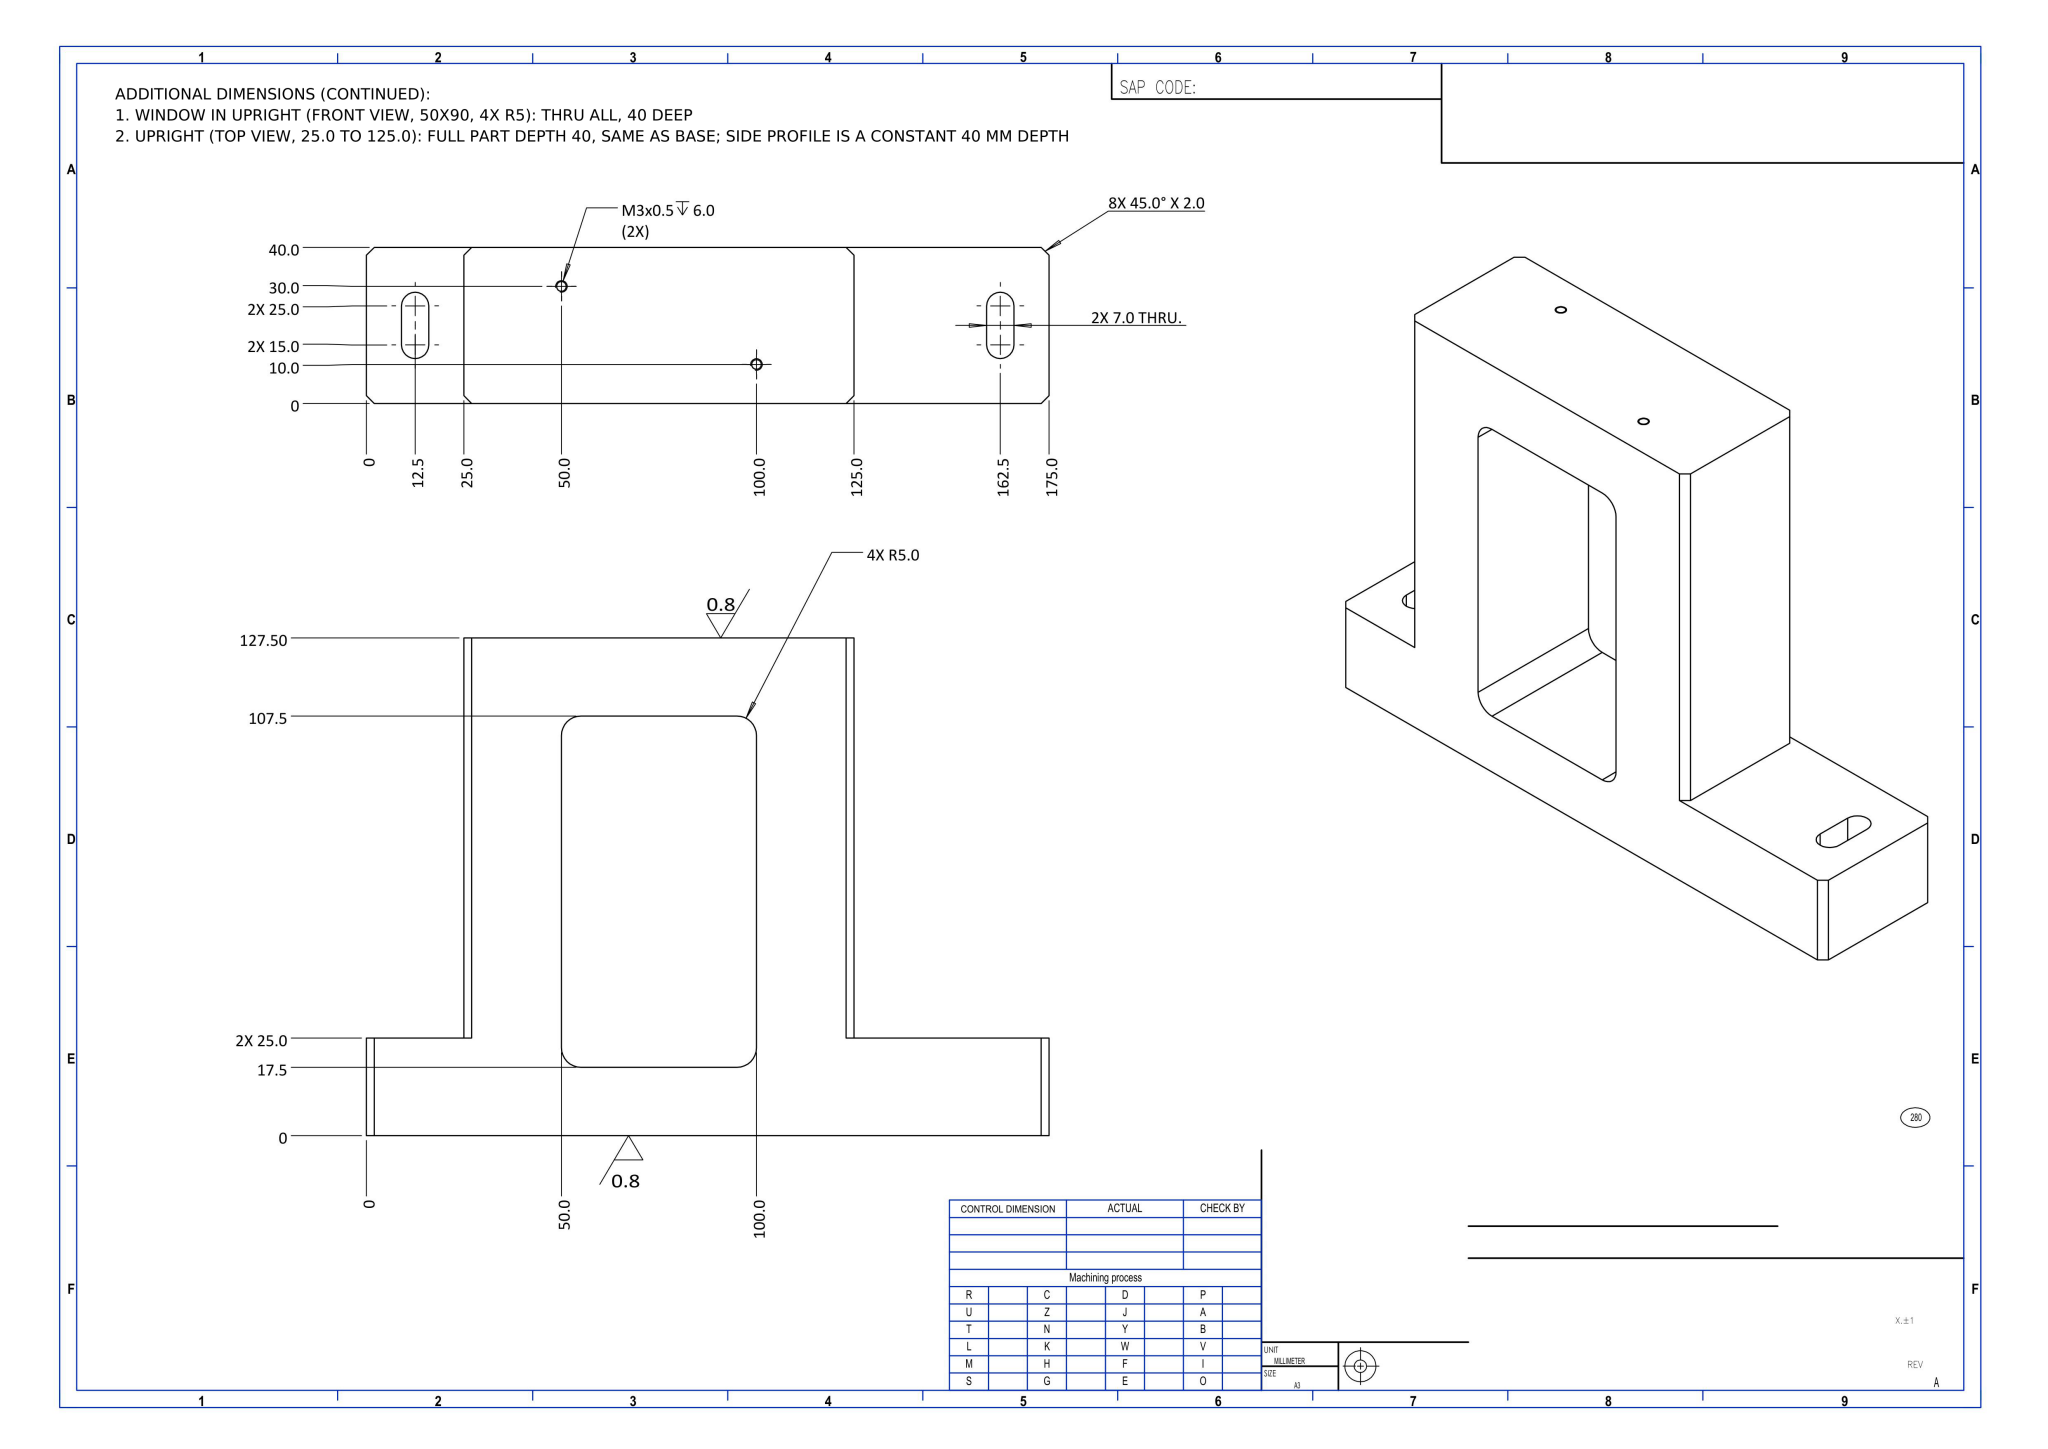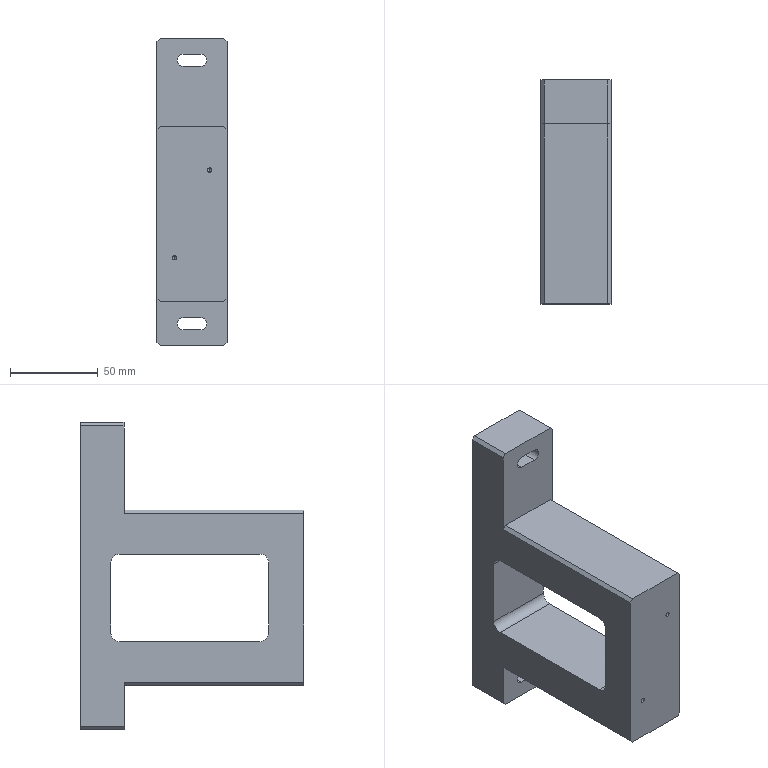Part | NX | mm | 1 solid | 42 faces | box 40 x 127.5 x 175 mm | volume 399289 mm3 | plane 26 | cylinder 12 | cone 4 | commonest cylinder face diameters 2.5 x4 7 x4 10 x4